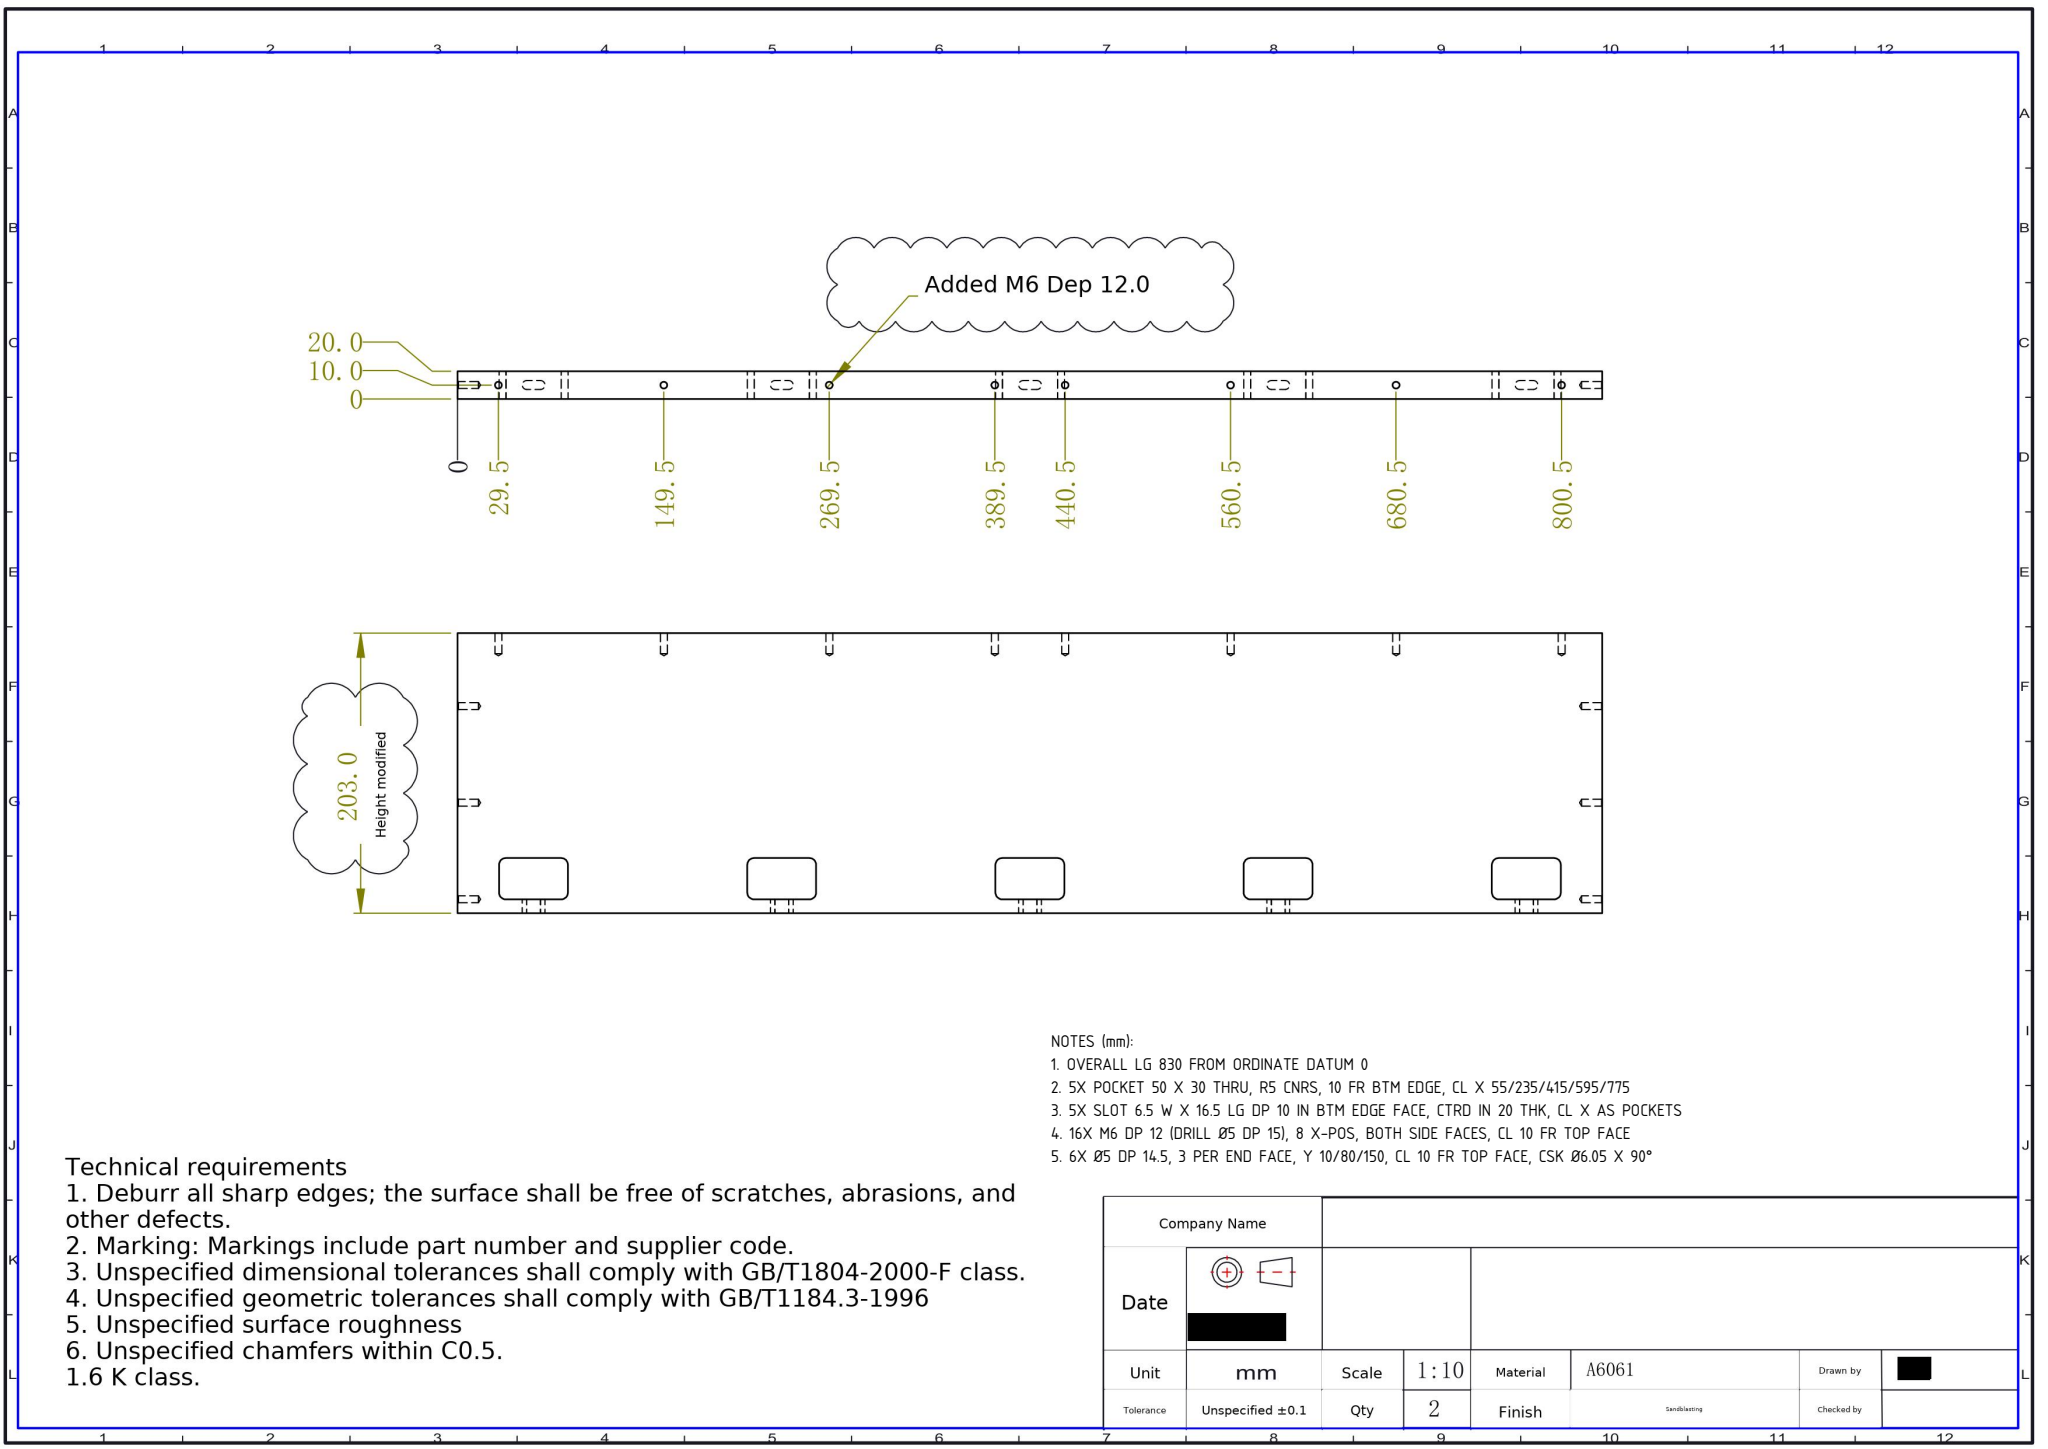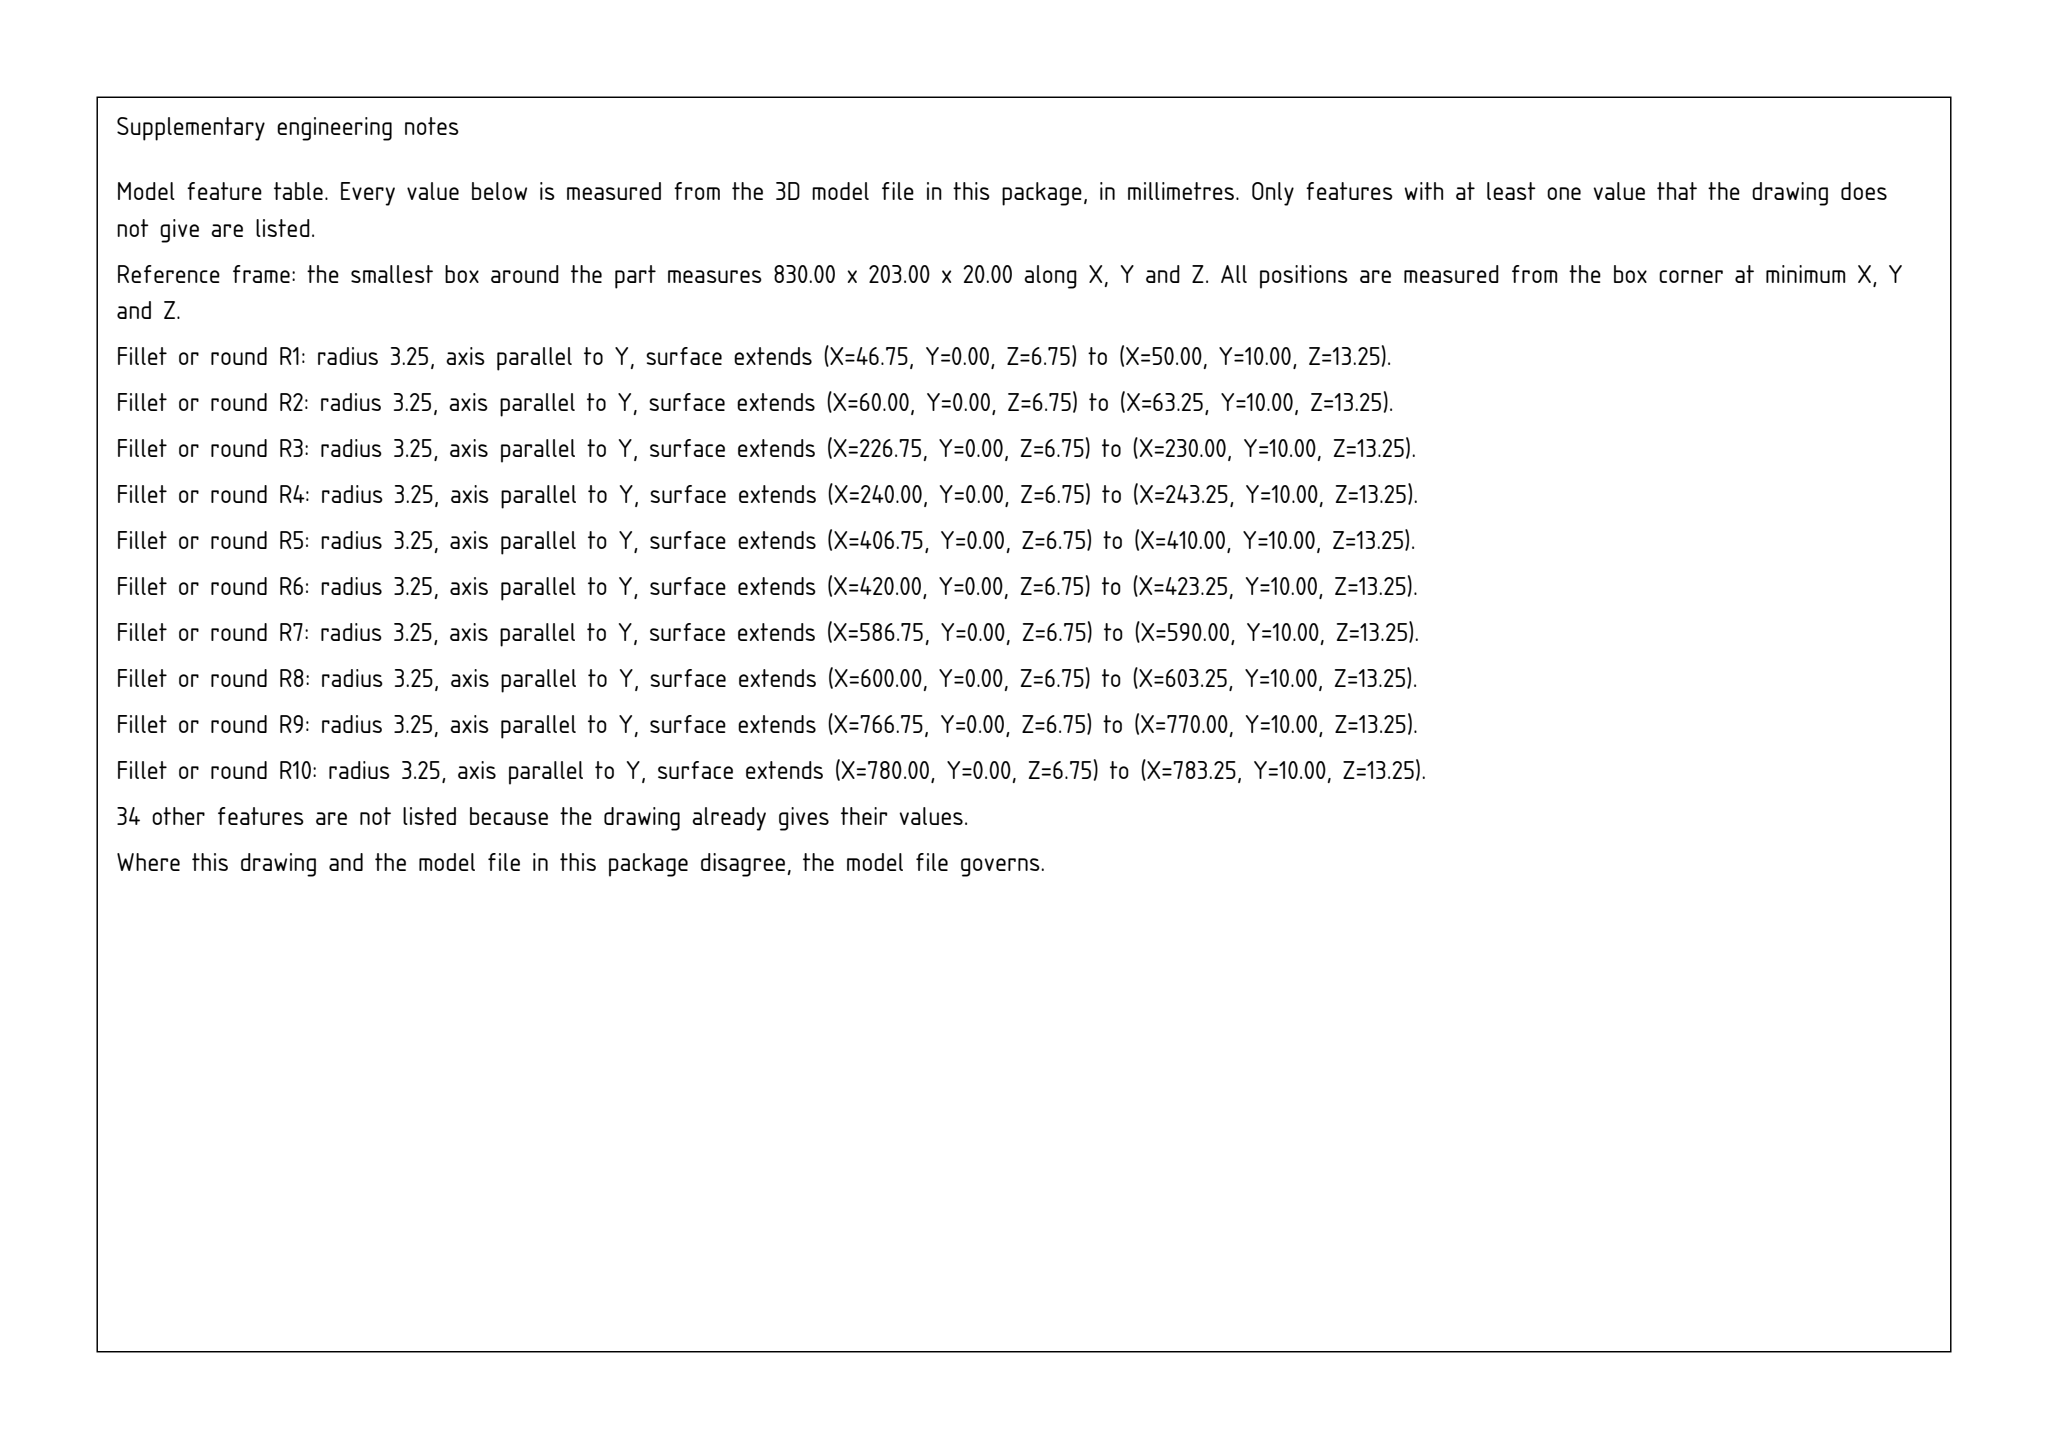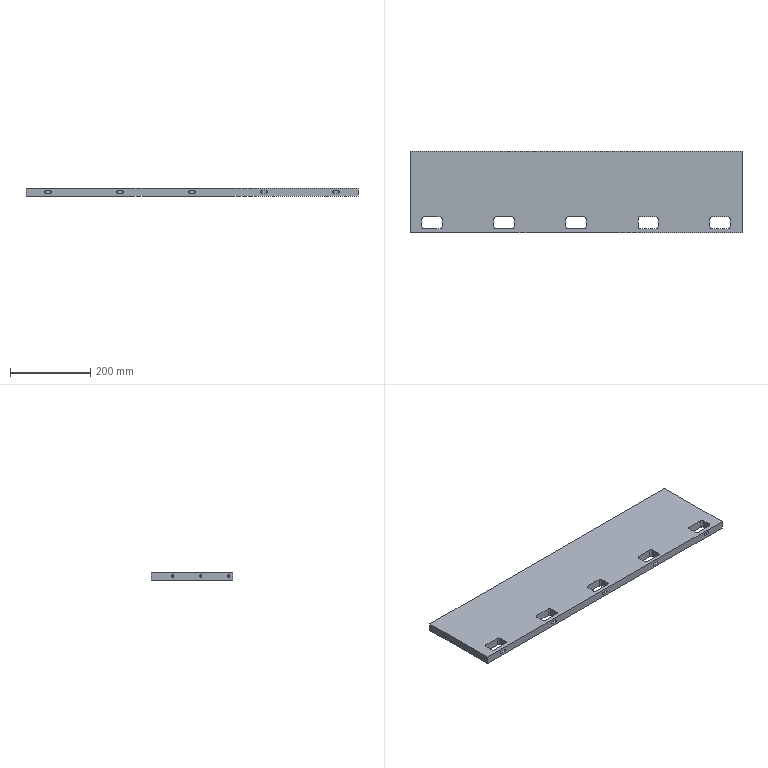Part | SolidWorks | mm | 1 solid | 134 faces | box 830 x 203 x 20 mm | volume 3212762 mm3 | cylinder 58 | cone 40 | plane 36 | commonest cylinder face diameters 5 x28 10 x20 6.5 x10
Drawing notes:
OVERALL LG 830 FROM ORDINATE DATUM 0 | from the solid: bbox_xyz X = 830.0; x planes at 0.0 and 830.0
5X POCKET 50 X 30 THRU, R5 CNRS, 10 FR BTM EDGE, CL X 55/235/415/595/775 | from the solid: x planes 30/80,210/260,390/440,570/620,750/800; y planes 10 & 40 (x5); Ø10 z-axis cyls L=20 at pocket cnrs; pitch 180
5X SLOT 6.5 W X 16.5 LG DP 10 IN BTM EDGE FACE, CTRD IN 20 THK, CL X AS POCKETS | from the solid: Ø6.5 y-axis cyls L10 at x=50/60,230/240,410/420,590/600,770/780, z=10; z planes 6.75 & 13.25 (x5)
16X M6 DP 12 (DRILL Ø5 DP 15), 8 X-POS, BOTH SIDE FACES, CL 10 FR TOP FACE | from the solid: Ø5 y-axis cyls L15 at X=29.5,149.5,269.5,389.5,440.5,560.5,680.5,800.5, 2 each; z=10 of 20 thk; 118 deg drill cones
6X Ø5 DP 14.5, 3 PER END FACE, Y 10/80/150, CL 10 FR TOP FACE, CSK Ø6.05 X 90° | from the solid: [5.0,'x',[null,10.0/80.0/150.0,10.0],14.48,4] at x=0 and x=830; cones [90.0,6.05] x12